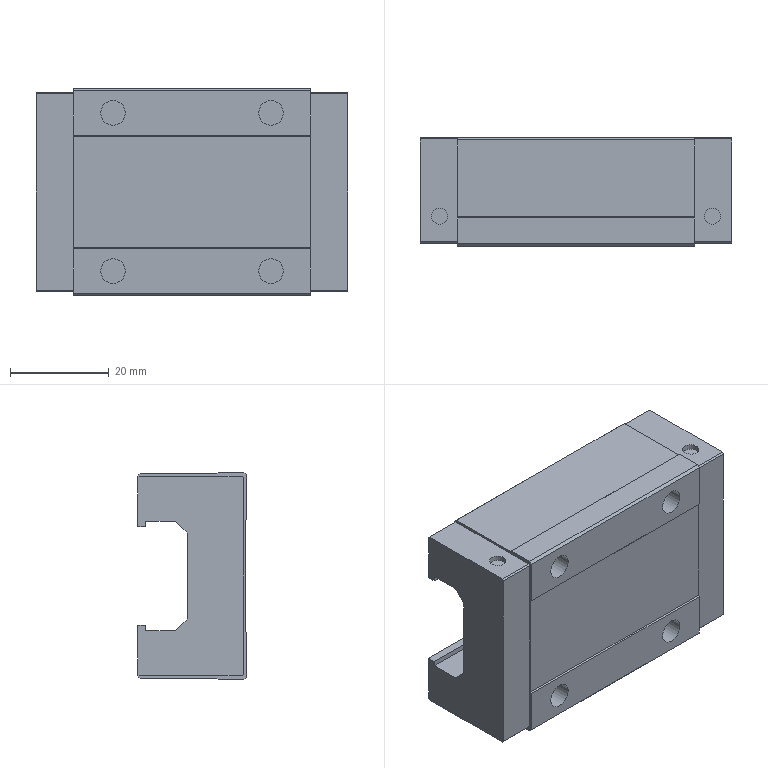Component | NX | SLIDER_2 | 1 solid | 60 faces | volume 42524 mm3 | plane 52 | cylinder 8 | commonest cylinder face diameters 3.3 x4 5 x4